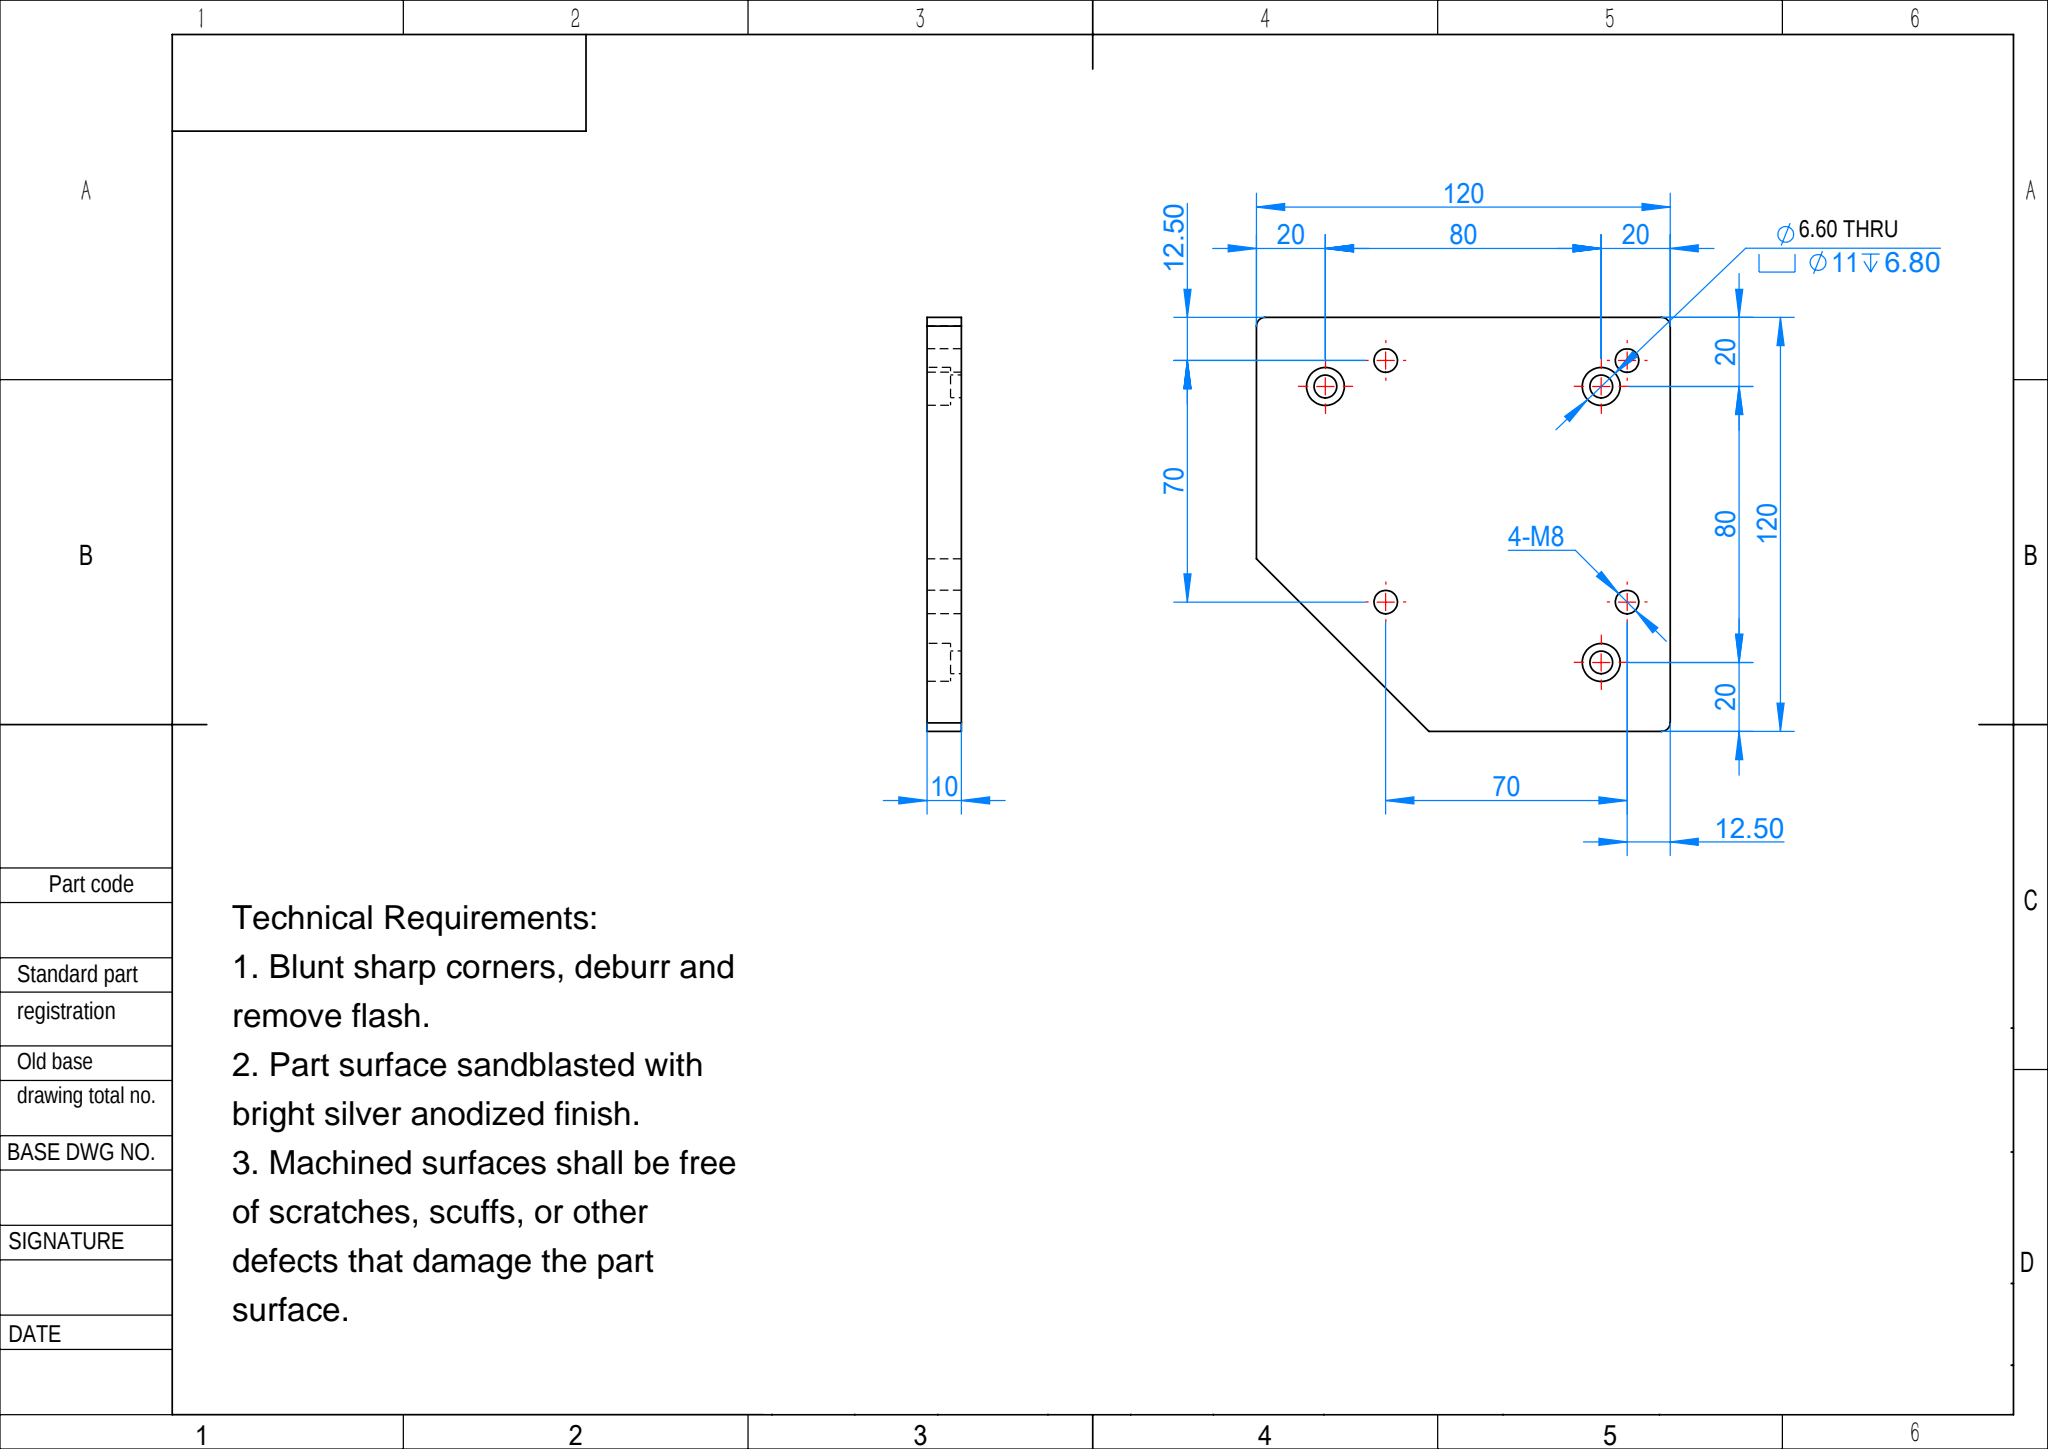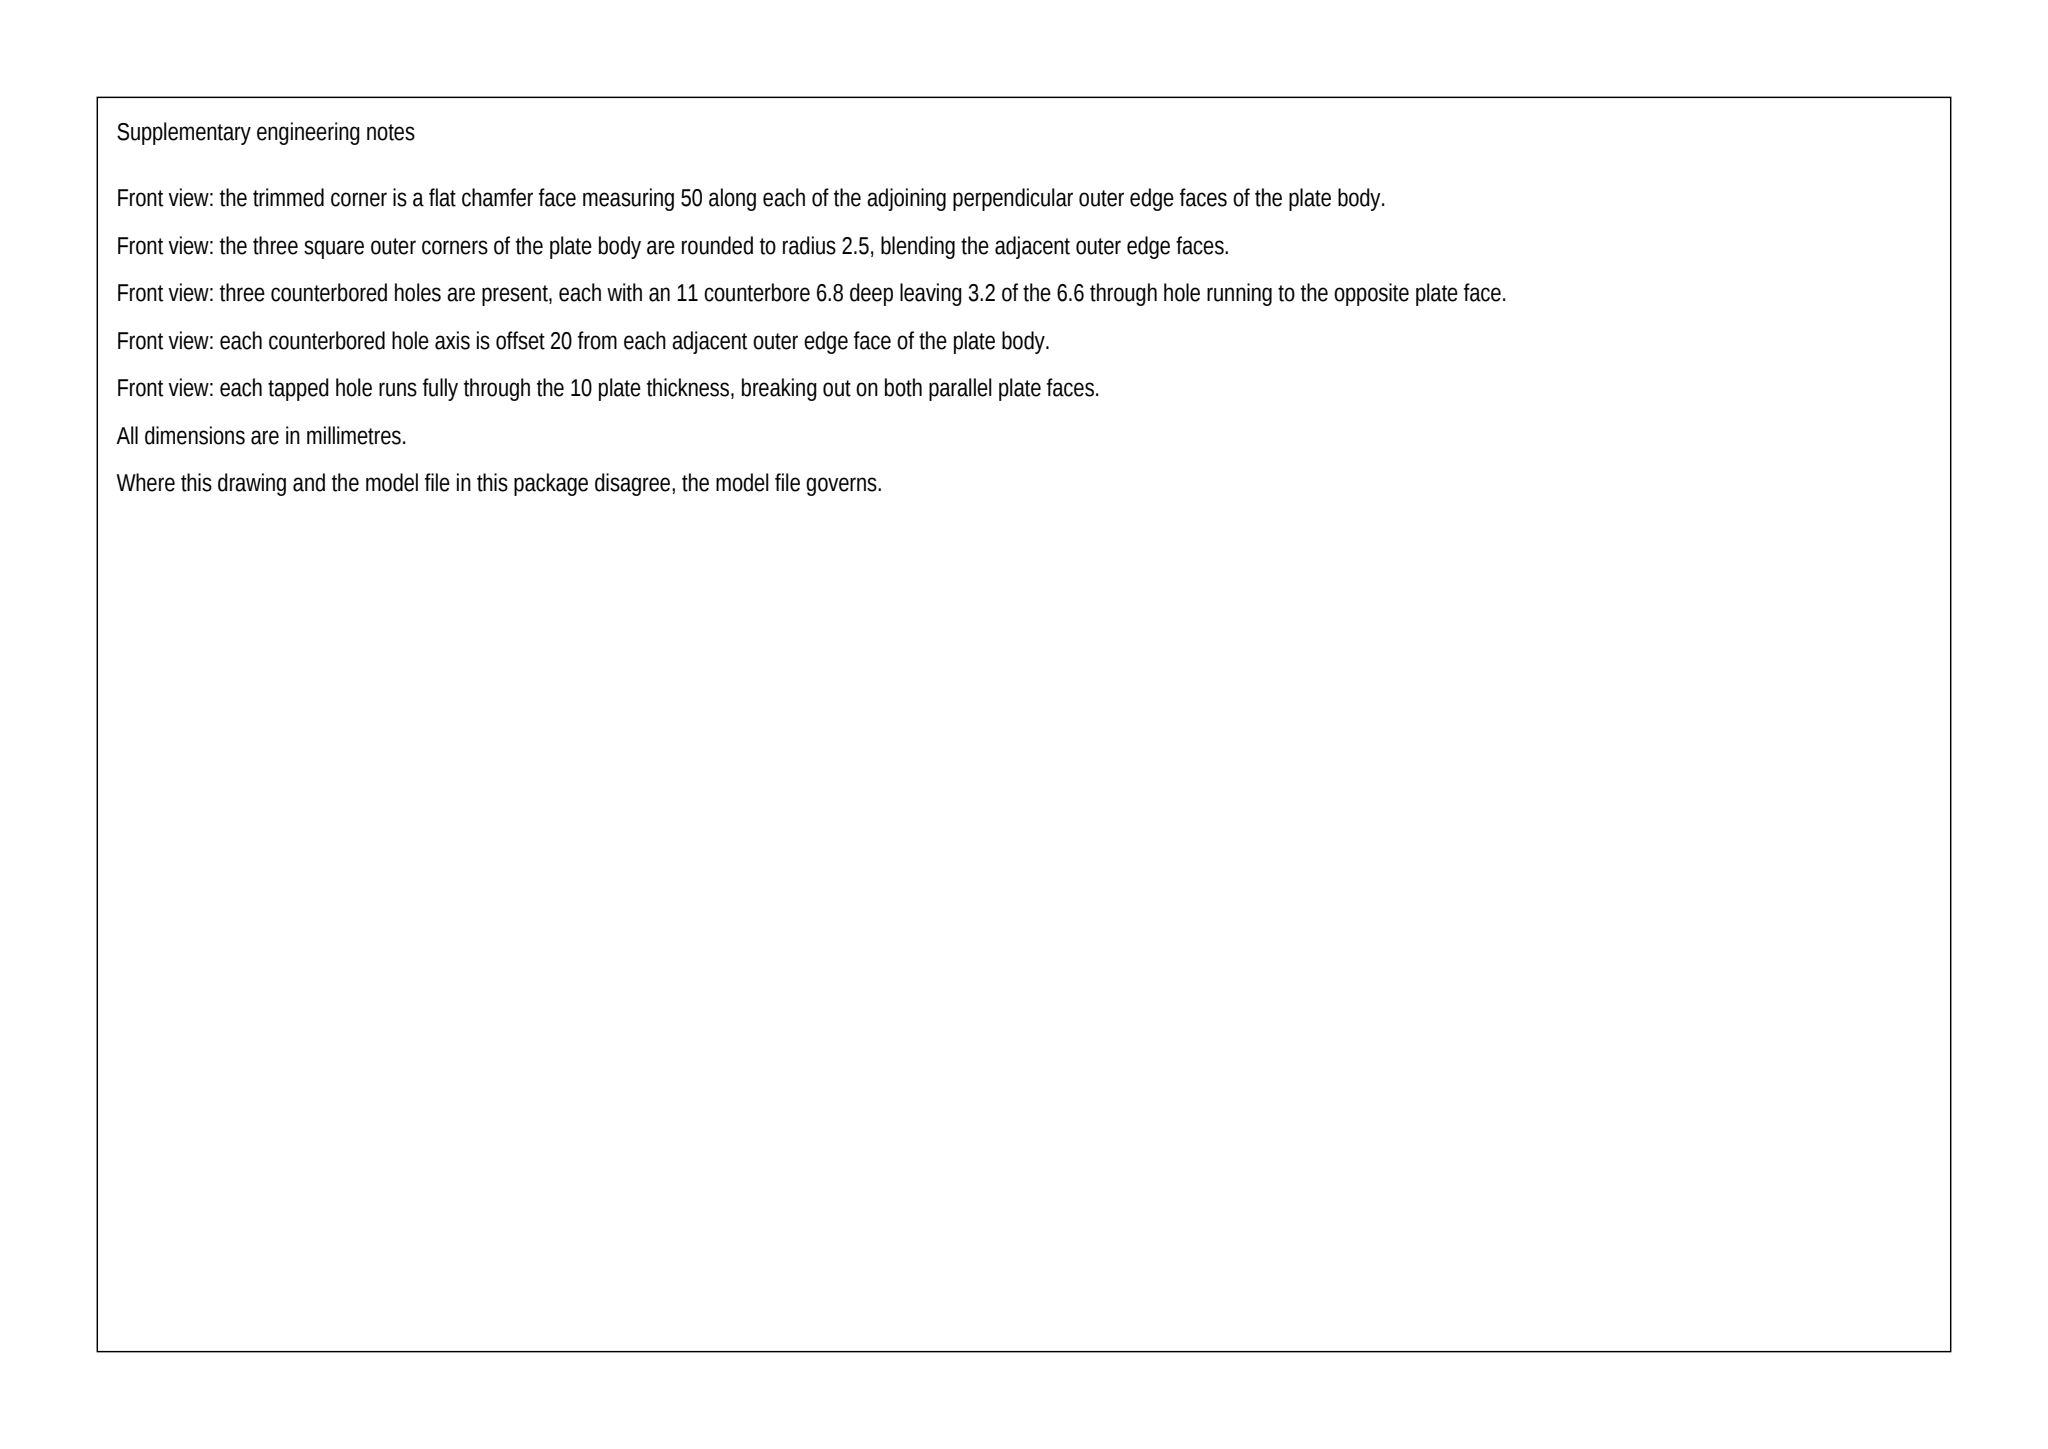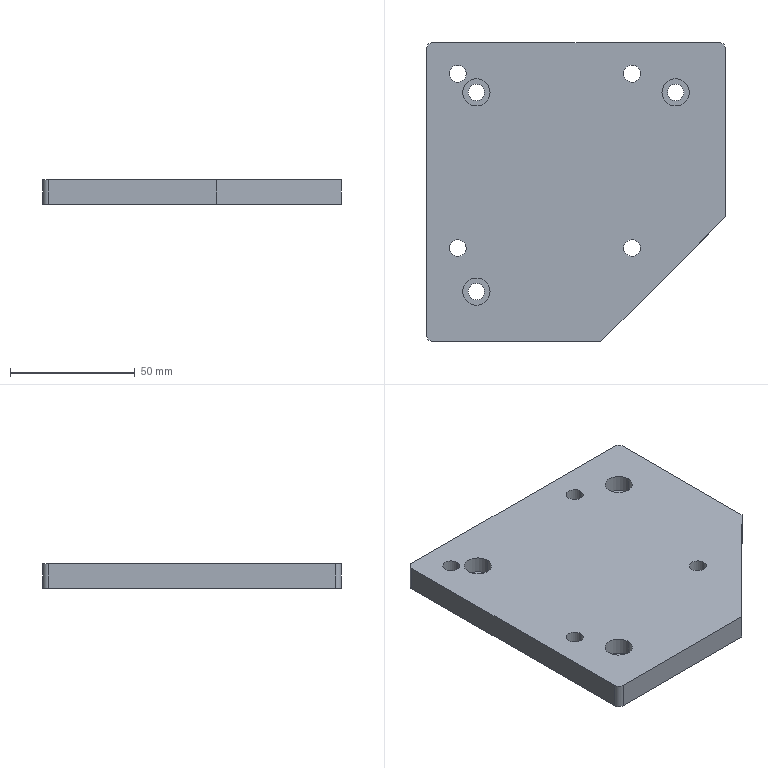Part | SolidWorks | mm | 1 solid | 33 faces | box 120 x 120 x 10 mm | volume 127740 mm3 | cylinder 23 | plane 10 | commonest cylinder face diameters 6.8 x8 6.6 x6 11 x6 5 x3
Drawing notes:
ANGLED CORNER CUT: 45° CHAMFER, 50 X 50 LEGS | from the solid: 120x120 bbox; corner at X120/Y0 has no R2.5 cyl, cut face at 45° joining edges 50 from that corner
Ø6.60 THRU, CBORE Ø11 DP 6.8 FROM TOP FACE | from the solid: Ø11 z-cyl length 6.8 with bottom plane z=3.2; Ø6.6 cyl z=0-3.2; plate 10 thk
3X Ø6.60 THRU, CBORE Ø11 DP 6.8 | from the solid: Ø11/Ø6.6 pairs at (20,20),(20,100),(100,100) = 3 places
UNSPECIFIED CORNER RADII R2.5 (3 PLCS) | from the solid: Ø5 z-cyls, full 10 length, at (2.5,2.5),(2.5,117.5),(117.5,117.5)
4-M8 THRU ALL (10 THK) | from the solid: Ø6.8 tap-drill z-cyls length 10 at (12.5,37.5),(12.5,107.5),(82.5,37.5),(82.5,107.5)